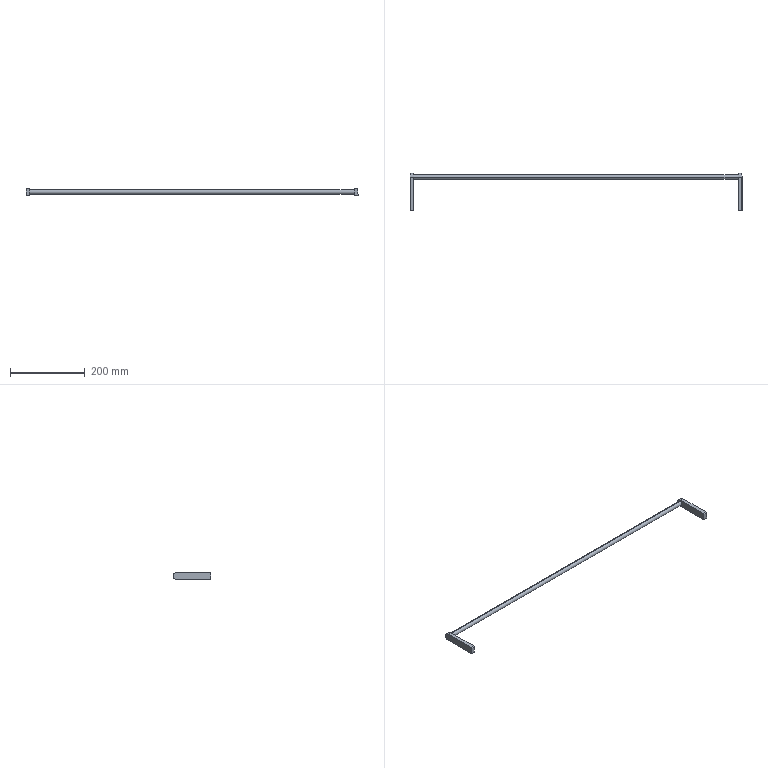Component | SolidWorks | D012-1 | 2 solids | 22 faces | box 889 x 100 x 20 mm | volume 137403 mm3 | plane 16 | cylinder 6 | commonest cylinder face diameters 12 x4 20 x2
build123d program:
from build123d import *

# Parameters (mm, degrees)
SKETCH1_W           = 100
SKETCH1_H           = 20
BOSS_EXTRUDE1_DEPTH = 10
FILLET1_RADIUS      = 10
FILLET1_LENGTH      = 10
SKETCH2_R           = 6
CUT_EXTRUDE1_DEPTH  = 2
SKETCH3_R           = 6
BOSS_EXTRUDE2_DEPTH = 871
BOSS_EXTRUDE3_START = 10
BOSS_EXTRUDE3_DEPTH = 10
CHAMFER1_SIZE       = 1
CHAMFER2_SIZE       = 1


with BuildPart() as part:
    # Sketch1 → Boss-Extrude1 (new body)
    with BuildSketch(Plane(origin=(0, 0, 0), x_dir=(1, 0, 0), z_dir=(0, 1, 0))):
        with Locations((50, 10)):
            Rectangle(SKETCH1_W, SKETCH1_H)
    extrude(amount=BOSS_EXTRUDE1_DEPTH)

    # Fillet1: full round fillet: the end face becomes a half cylinder, R = half its width
    fillet1_face = Plane((100, 5, -10), x_dir=(0, 1, 0), z_dir=(1, 0, 0))  # on the end face: x along it, z out of the body
    fillet1_slab = fillet1_face.offset(-FILLET1_RADIUS / 2) * Box(FILLET1_LENGTH, 2 * FILLET1_RADIUS, FILLET1_RADIUS, mode=Mode.PRIVATE)  # the body's end, R deep
    fillet1_round = Plane((90, 5, -10), x_dir=(1, 0, 0), z_dir=(0, 1, 0)) * Cylinder(FILLET1_RADIUS, FILLET1_LENGTH, mode=Mode.PRIVATE)  # its axis R under the face
    add(fillet1_slab - fillet1_round, mode=Mode.SUBTRACT)

    # Sketch2 → Cut-Extrude1 (cut)
    with BuildSketch(Plane(origin=(0, 10, 0), x_dir=(1, 0, 0), z_dir=(0, 1, 0))):
        with Locations(Location((90, 10, 0), (0, 0, 270))):
            Circle(SKETCH2_R)
    extrude(amount=-CUT_EXTRUDE1_DEPTH, mode=Mode.SUBTRACT)

    # Chamfer1
    chamfer1_edges = [part.edges().sort_by_distance(p)[0] for p in [
        (0, 5, -20),
        (0, 5, 0),
    ]]
    chamfer(chamfer1_edges, length=CHAMFER1_SIZE)


with BuildPart() as body_2:
    # Sketch3 → Boss-Extrude2 (new body)
    with BuildSketch(Plane(origin=(0, 8, 0), x_dir=(1, 0, 0), z_dir=(0, 1, 0))):
        with Locations(Location((90, 10, 0), (0, 0, 90))):
            Circle(SKETCH3_R)
    extrude(amount=BOSS_EXTRUDE2_DEPTH)

    # Sketch4 → Boss-Extrude3 (add)
    with BuildSketch(Plane(origin=(0, 879, 0), x_dir=(1, 0, 0), z_dir=(0, 1, 0)).offset(BOSS_EXTRUDE3_START)):
        with BuildLine():
            Line((0, 0), (90, 0))
            ThreePointArc((90, 0), (100, 10), (90, 20))
            Line((90, 20), (0, 20))
            Line((0, 20), (0, 0))
        make_face()
    extrude(amount=-BOSS_EXTRUDE3_DEPTH)

    # Chamfer2
    chamfer2_edges = [body_2.edges().sort_by_distance(p)[0] for p in [
        (0, 884, -20),
        (0, 884, 0),
    ]]
    chamfer(chamfer2_edges, length=CHAMFER2_SIZE)


solid = Compound([part.part, body_2.part])

# Placed as in the assembly
solid = solid.moved(Location((879, -35, 32.732), (0, 0, 90)))
STEP:
#1=CARTESIAN_POINT('',(-0.,2.165,1.131));
#2=VERTEX_POINT('',#1);
#3=CARTESIAN_POINT('',(-0.,2.165,0.6587));
#4=VERTEX_POINT('',#3);
#5=CARTESIAN_POINT('',(-0.,2.165,0.895));
#6=DIRECTION('',(-1.,-0.,-0.));
#7=DIRECTION('',(-0.,-0.,1.));
#8=AXIS2_PLACEMENT_3D('',#5,#6,#7);
#9=CIRCLE('',#8,0.2362);
#10=EDGE_CURVE('',#2,#4,#9,.T.);
#11=ORIENTED_EDGE('',*,*,#10,.F.);
#12=CARTESIAN_POINT('',(34.291,2.165,1.131));
#13=VERTEX_POINT('',#12);
#14=CARTESIAN_POINT('',(-0.,2.165,1.131));
#15=DIRECTION('',(1.,0.,0.));
#16=VECTOR('',#15,39.37);
#17=LINE('',#14,#16);
#18=EDGE_CURVE('',#2,#13,#17,.T.);
#19=ORIENTED_EDGE('',*,*,#18,.T.);
#20=CARTESIAN_POINT('',(34.291,2.165,0.6587));
#21=VERTEX_POINT('',#20);
#22=CARTESIAN_POINT('',(34.291,2.165,0.895));
#23=DIRECTION('',(-1.,-0.,-0.));
#24=DIRECTION('',(0.,-0.,1.));
#25=AXIS2_PLACEMENT_3D('',#22,#23,#24);
#26=CIRCLE('',#25,0.2362);
#27=EDGE_CURVE('',#13,#21,#26,.T.);
#28=ORIENTED_EDGE('',*,*,#27,.T.);
#29=CARTESIAN_POINT('',(-0.,2.165,0.6587));
#30=DIRECTION('',(1.,0.,0.));
#31=VECTOR('',#30,39.37);
#32=LINE('',#29,#31);
#33=EDGE_CURVE('',#4,#21,#32,.T.);
#34=ORIENTED_EDGE('',*,*,#33,.F.);
#35=EDGE_LOOP('',(#11,#19,#28,#34));
#36=FACE_OUTER_BOUND('',#35,.T.);
#37=CARTESIAN_POINT('',(-0.,2.165,0.895));
#38=DIRECTION('',(1.,0.,0.));
#39=DIRECTION('',(0.,0.,-1.));
#40=AXIS2_PLACEMENT_3D('',#37,#38,#39);
#41=CYLINDRICAL_SURFACE('',#40,0.2362);
#42=ADVANCED_FACE('',(#36),#41,.T.);
#43=ORIENTED_EDGE('',*,*,#18,.F.);
#44=CARTESIAN_POINT('',(-0.,2.165,0.895));
#45=DIRECTION('',(-1.,-0.,-0.));
#46=DIRECTION('',(-0.,-0.,1.));
#47=AXIS2_PLACEMENT_3D('',#44,#45,#46);
#48=CIRCLE('',#47,0.2362);
#49=EDGE_CURVE('',#4,#2,#48,.T.);
#50=ORIENTED_EDGE('',*,*,#49,.F.);
#51=ORIENTED_EDGE('',*,*,#33,.T.);
#52=CARTESIAN_POINT('',(34.291,2.165,0.895));
#53=DIRECTION('',(-1.,-0.,-0.));
#54=DIRECTION('',(0.,-0.,1.));
#55=AXIS2_PLACEMENT_3D('',#52,#53,#54);
#56=CIRCLE('',#55,0.2362);
#57=EDGE_CURVE('',#21,#13,#56,.T.);
#58=ORIENTED_EDGE('',*,*,#57,.T.);
#59=EDGE_LOOP('',(#43,#50,#51,#58));
#60=FACE_OUTER_BOUND('',#59,.T.);
#61=CARTESIAN_POINT('',(-0.,2.165,0.895));
#62=DIRECTION('',(1.,0.,0.));
#63=DIRECTION('',(0.,0.,-1.));
#64=AXIS2_PLACEMENT_3D('',#61,#62,#63);
#65=CYLINDRICAL_SURFACE('',#64,0.2362);
#66=ADVANCED_FACE('',(#60),#65,.T.);
#67=ORIENTED_EDGE('',*,*,#57,.F.);
#68=ORIENTED_EDGE('',*,*,#27,.F.);
#69=EDGE_LOOP('',(#67,#68));
#70=FACE_OUTER_BOUND('',#69,.T.);
#71=CARTESIAN_POINT('',(34.291,2.165,0.895));
#72=DIRECTION('',(-1.,-0.,-0.));
#73=DIRECTION('',(-0.,-0.,1.));
#74=AXIS2_PLACEMENT_3D('',#71,#72,#73);
#75=PLANE('',#74);
#76=ADVANCED_FACE('',(#70),#75,.F.);
#77=CARTESIAN_POINT('',(-0.,-1.378,0.5406));
#78=VERTEX_POINT('',#77);
#79=CARTESIAN_POINT('',(-0.,-1.378,1.249));
#80=VERTEX_POINT('',#79);
#81=CARTESIAN_POINT('',(-0.,-1.378,0.5013));
#82=DIRECTION('',(-0.,-0.,1.));
#83=VECTOR('',#82,39.37);
#84=LINE('',#81,#83);
#85=EDGE_CURVE('',#78,#80,#84,.T.);
#86=ORIENTED_EDGE('',*,*,#85,.T.);
#87=CARTESIAN_POINT('',(-0.3937,-1.378,1.249));
#88=VERTEX_POINT('',#87);
#89=CARTESIAN_POINT('',(-0.3937,-1.378,1.249));
#90=DIRECTION('',(-1.,-0.,-0.));
#91=VECTOR('',#90,39.37);
#92=LINE('',#89,#91);
#93=EDGE_CURVE('',#80,#88,#92,.T.);
#94=ORIENTED_EDGE('',*,*,#93,.T.);
#95=CARTESIAN_POINT('',(-0.3937,-1.378,0.5406));
#96=VERTEX_POINT('',#95);
#97=CARTESIAN_POINT('',(-0.3937,-1.378,0.5013));
#98=DIRECTION('',(-0.,-0.,1.));
#99=VECTOR('',#98,39.37);
#100=LINE('',#97,#99);
#101=EDGE_CURVE('',#96,#88,#100,.T.);
#102=ORIENTED_EDGE('',*,*,#101,.F.);
#103=CARTESIAN_POINT('',(-0.3937,-1.378,0.5406));
#104=DIRECTION('',(1.,0.,0.));
#105=VECTOR('',#104,39.37);
#106=LINE('',#103,#105);
#107=EDGE_CURVE('',#96,#78,#106,.T.);
#108=ORIENTED_EDGE('',*,*,#107,.T.);
#109=EDGE_LOOP('',(#86,#94,#102,#108));
#110=FACE_OUTER_BOUND('',#109,.T.);
#111=CARTESIAN_POINT('',(-0.3937,-1.378,0.5013));
#112=DIRECTION('',(-0.,1.,0.));
#113=DIRECTION('',(0.,0.,-1.));
#114=AXIS2_PLACEMENT_3D('',#111,#112,#113);
#115=PLANE('',#114);
#116=ADVANCED_FACE('',(#110),#115,.F.);
#117=CARTESIAN_POINT('',(-0.3937,-1.339,1.289));
#118=VERTEX_POINT('',#117);
#119=CARTESIAN_POINT('',(-0.3937,2.165,1.289));
#120=VERTEX_POINT('',#119);
#121=CARTESIAN_POINT('',(-0.3937,-1.378,1.289));
#122=DIRECTION('',(-0.,1.,0.));
#123=VECTOR('',#122,39.37);
#124=LINE('',#121,#123);
#125=EDGE_CURVE('',#118,#120,#124,.T.);
#126=ORIENTED_EDGE('',*,*,#125,.F.);
#127=CARTESIAN_POINT('',(-0.,-1.339,1.289));
#128=VERTEX_POINT('',#127);
#129=CARTESIAN_POINT('',(-0.3937,-1.339,1.289));
#130=DIRECTION('',(1.,0.,0.));
#131=VECTOR('',#130,39.37);
#132=LINE('',#129,#131);
#133=EDGE_CURVE('',#118,#128,#132,.T.);
#134=ORIENTED_EDGE('',*,*,#133,.T.);
#135=CARTESIAN_POINT('',(-0.,2.165,1.289));
#136=VERTEX_POINT('',#135);
#137=CARTESIAN_POINT('',(-0.,-1.378,1.289));
#138=DIRECTION('',(-0.,1.,0.));
#139=VECTOR('',#138,39.37);
#140=LINE('',#137,#139);
#141=EDGE_CURVE('',#128,#136,#140,.T.);
#142=ORIENTED_EDGE('',*,*,#141,.T.);
#143=CARTESIAN_POINT('',(-0.3937,2.165,1.289));
#144=DIRECTION('',(1.,0.,0.));
#145=VECTOR('',#144,39.37);
#146=LINE('',#143,#145);
#147=EDGE_CURVE('',#120,#136,#146,.T.);
#148=ORIENTED_EDGE('',*,*,#147,.F.);
#149=EDGE_LOOP('',(#126,#134,#142,#148));
#150=FACE_OUTER_BOUND('',#149,.T.);
#151=CARTESIAN_POINT('',(-0.3937,-1.378,1.289));
#152=DIRECTION('',(0.,0.,-1.));
#153=DIRECTION('',(0.,-1.,-0.));
#154=AXIS2_PLACEMENT_3D('',#151,#152,#153);
#155=PLANE('',#154);
#156=ADVANCED_FACE('',(#150),#155,.F.);
#157=CARTESIAN_POINT('',(-0.,2.165,0.5013));
#158=VERTEX_POINT('',#157);
#159=CARTESIAN_POINT('',(-0.,2.165,0.895));
#160=DIRECTION('',(-1.,-0.,-0.));
#161=DIRECTION('',(-0.,-0.,1.));
#162=AXIS2_PLACEMENT_3D('',#159,#160,#161);
#163=CIRCLE('',#162,0.3937);
#164=EDGE_CURVE('',#136,#158,#163,.T.);
#165=ORIENTED_EDGE('',*,*,#164,.T.);
#166=CARTESIAN_POINT('',(-0.3937,2.165,0.5013));
#167=VERTEX_POINT('',#166);
#168=CARTESIAN_POINT('',(-0.3937,2.165,0.5013));
#169=DIRECTION('',(1.,0.,0.));
#170=VECTOR('',#169,39.37);
#171=LINE('',#168,#170);
#172=EDGE_CURVE('',#167,#158,#171,.T.);
#173=ORIENTED_EDGE('',*,*,#172,.F.);
#174=CARTESIAN_POINT('',(-0.3937,2.165,0.895));
#175=DIRECTION('',(-1.,-0.,-0.));
#176=DIRECTION('',(-0.,-0.,1.));
#177=AXIS2_PLACEMENT_3D('',#174,#175,#176);
#178=CIRCLE('',#177,0.3937);
#179=EDGE_CURVE('',#120,#167,#178,.T.);
#180=ORIENTED_EDGE('',*,*,#179,.F.);
#181=ORIENTED_EDGE('',*,*,#147,.T.);
#182=EDGE_LOOP('',(#165,#173,#180,#181));
#183=FACE_OUTER_BOUND('',#182,.T.);
#184=CARTESIAN_POINT('',(-0.3937,2.165,0.895));
#185=DIRECTION('',(1.,0.,0.));
#186=DIRECTION('',(0.,0.,-1.));
#187=AXIS2_PLACEMENT_3D('',#184,#185,#186);
#188=CYLINDRICAL_SURFACE('',#187,0.3937);
#189=ADVANCED_FACE('',(#183),#188,.T.);
#190=CARTESIAN_POINT('',(-0.,-1.339,0.5013));
#191=VERTEX_POINT('',#190);
#192=CARTESIAN_POINT('',(-0.,2.165,0.5013));
#193=DIRECTION('',(0.,-1.,-0.));
#194=VECTOR('',#193,39.37);
#195=LINE('',#192,#194);
#196=EDGE_CURVE('',#158,#191,#195,.T.);
#197=ORIENTED_EDGE('',*,*,#196,.T.);
#198=CARTESIAN_POINT('',(-0.3937,-1.339,0.5013));
#199=VERTEX_POINT('',#198);
#200=CARTESIAN_POINT('',(-0.3937,-1.339,0.5013));
#201=DIRECTION('',(-1.,-0.,-0.));
#202=VECTOR('',#201,39.37);
#203=LINE('',#200,#202);
#204=EDGE_CURVE('',#191,#199,#203,.T.);
#205=ORIENTED_EDGE('',*,*,#204,.T.);
#206=CARTESIAN_POINT('',(-0.3937,2.165,0.5013));
#207=DIRECTION('',(0.,-1.,-0.));
#208=VECTOR('',#207,39.37);
#209=LINE('',#206,#208);
#210=EDGE_CURVE('',#167,#199,#209,.T.);
#211=ORIENTED_EDGE('',*,*,#210,.F.);
#212=ORIENTED_EDGE('',*,*,#172,.T.);
#213=EDGE_LOOP('',(#197,#205,#211,#212));
#214=FACE_OUTER_BOUND('',#213,.T.);
#215=CARTESIAN_POINT('',(-0.3937,2.165,0.5013));
#216=DIRECTION('',(-0.,-0.,1.));
#217=DIRECTION('',(-0.,1.,0.));
#218=AXIS2_PLACEMENT_3D('',#215,#216,#217);
#219=PLANE('',#218);
#220=ADVANCED_FACE('',(#214),#219,.F.);
#221=ORIENTED_EDGE('',*,*,#101,.T.);
#222=CARTESIAN_POINT('',(-0.3937,0.2165,2.844));
#223=DIRECTION('',(-0.,0.7071,0.7071));
#224=VECTOR('',#223,39.37);
#225=LINE('',#222,#224);
#226=EDGE_CURVE('',#88,#118,#225,.T.);
#227=ORIENTED_EDGE('',*,*,#226,.T.);
#228=ORIENTED_EDGE('',*,*,#125,.T.);
#229=ORIENTED_EDGE('',*,*,#179,.T.);
#230=ORIENTED_EDGE('',*,*,#210,.T.);
#231=CARTESIAN_POINT('',(-0.3937,0.2165,-1.054));
#232=DIRECTION('',(-0.,-0.7071,0.7071));
#233=VECTOR('',#232,39.37);
#234=LINE('',#231,#233);
#235=EDGE_CURVE('',#199,#96,#234,.T.);
#236=ORIENTED_EDGE('',*,*,#235,.T.);
#237=EDGE_LOOP('',(#221,#227,#228,#229,#230,#236));
#238=FACE_OUTER_BOUND('',#237,.T.);
#239=CARTESIAN_POINT('',(-0.3937,2.165,0.895));
#240=DIRECTION('',(-1.,-0.,-0.));
#241=DIRECTION('',(-0.,-0.,1.));
#242=AXIS2_PLACEMENT_3D('',#239,#240,#241);
#243=PLANE('',#242);
#244=ADVANCED_FACE('',(#238),#243,.T.);
#245=ORIENTED_EDGE('',*,*,#49,.T.);
#246=ORIENTED_EDGE('',*,*,#10,.T.);
#247=EDGE_LOOP('',(#245,#246));
#248=FACE_BOUND('',#247,.T.);
#249=ORIENTED_EDGE('',*,*,#141,.F.);
#250=CARTESIAN_POINT('',(-0.,-1.339,1.289));
#251=DIRECTION('',(0.,-0.7071,-0.7071));
#252=VECTOR('',#251,39.37);
#253=LINE('',#250,#252);
#254=EDGE_CURVE('',#128,#80,#253,.T.);
#255=ORIENTED_EDGE('',*,*,#254,.T.);
#256=ORIENTED_EDGE('',*,*,#85,.F.);
#257=CARTESIAN_POINT('',(-0.,-1.378,0.5406));
#258=DIRECTION('',(0.,0.7071,-0.7071));
#259=VECTOR('',#258,39.37);
#260=LINE('',#257,#259);
#261=EDGE_CURVE('',#78,#191,#260,.T.);
#262=ORIENTED_EDGE('',*,*,#261,.T.);
#263=ORIENTED_EDGE('',*,*,#196,.F.);
#264=ORIENTED_EDGE('',*,*,#164,.F.);
#265=EDGE_LOOP('',(#249,#255,#256,#262,#263,#264));
#266=FACE_OUTER_BOUND('',#265,.T.);
#267=CARTESIAN_POINT('',(-0.,2.165,0.895));
#268=DIRECTION('',(-1.,-0.,-0.));
#269=DIRECTION('',(-0.,-0.,1.));
#270=AXIS2_PLACEMENT_3D('',#267,#268,#269);
#271=PLANE('',#270);
#272=ADVANCED_FACE('',(#248,#266),#271,.F.);
#273=ORIENTED_EDGE('',*,*,#226,.F.);
#274=ORIENTED_EDGE('',*,*,#93,.F.);
#275=ORIENTED_EDGE('',*,*,#254,.F.);
#276=ORIENTED_EDGE('',*,*,#133,.F.);
#277=EDGE_LOOP('',(#273,#274,#275,#276));
#278=FACE_OUTER_BOUND('',#277,.T.);
#279=CARTESIAN_POINT('',(-0.3937,-1.339,1.289));
#280=DIRECTION('',(0.,0.7071,-0.7071));
#281=DIRECTION('',(1.,0.,0.));
#282=AXIS2_PLACEMENT_3D('',#279,#280,#281);
#283=PLANE('',#282);
#284=ADVANCED_FACE('',(#278),#283,.F.);
#285=ORIENTED_EDGE('',*,*,#235,.F.);
#286=ORIENTED_EDGE('',*,*,#204,.F.);
#287=ORIENTED_EDGE('',*,*,#261,.F.);
#288=ORIENTED_EDGE('',*,*,#107,.F.);
#289=EDGE_LOOP('',(#285,#286,#287,#288));
#290=FACE_OUTER_BOUND('',#289,.T.);
#291=CARTESIAN_POINT('',(-0.3937,-1.378,0.5406));
#292=DIRECTION('',(-0.,0.7071,0.7071));
#293=DIRECTION('',(1.,0.,0.));
#294=AXIS2_PLACEMENT_3D('',#291,#292,#293);
#295=PLANE('',#294);
#296=ADVANCED_FACE('',(#290),#295,.F.);
#297=CLOSED_SHELL('',(#42,#66,#76,#116,#156,#189,#220,#244,#272,#284,#296));
#298=MANIFOLD_SOLID_BREP('',#297);
#299=CARTESIAN_POINT('',(34.291,2.165,0.6587));
#300=VERTEX_POINT('',#299);
#301=CARTESIAN_POINT('',(34.291,2.165,1.131));
#302=VERTEX_POINT('',#301);
#303=CARTESIAN_POINT('',(34.291,2.165,0.895));
#304=DIRECTION('',(-1.,-0.,-0.));
#305=DIRECTION('',(0.,-0.,1.));
#306=AXIS2_PLACEMENT_3D('',#303,#304,#305);
#307=CIRCLE('',#306,0.2362);
#308=EDGE_CURVE('',#300,#302,#307,.T.);
#309=ORIENTED_EDGE('',*,*,#308,.F.);
#310=CARTESIAN_POINT('',(34.213,2.165,0.6587));
#311=VERTEX_POINT('',#310);
#312=CARTESIAN_POINT('',(34.291,2.165,0.6587));
#313=DIRECTION('',(-1.,-0.,-0.));
#314=VECTOR('',#313,39.37);
#315=LINE('',#312,#314);
#316=EDGE_CURVE('',#300,#311,#315,.T.);
#317=ORIENTED_EDGE('',*,*,#316,.T.);
#318=CARTESIAN_POINT('',(34.213,2.165,1.131));
#319=VERTEX_POINT('',#318);
#320=CARTESIAN_POINT('',(34.213,2.165,0.895));
#321=DIRECTION('',(-1.,-0.,-0.));
#322=DIRECTION('',(0.,-0.,1.));
#323=AXIS2_PLACEMENT_3D('',#320,#321,#322);
#324=CIRCLE('',#323,0.2362);
#325=EDGE_CURVE('',#311,#319,#324,.T.);
#326=ORIENTED_EDGE('',*,*,#325,.T.);
#327=CARTESIAN_POINT('',(34.291,2.165,1.131));
#328=DIRECTION('',(-1.,-0.,-0.));
#329=VECTOR('',#328,39.37);
#330=LINE('',#327,#329);
#331=EDGE_CURVE('',#302,#319,#330,.T.);
#332=ORIENTED_EDGE('',*,*,#331,.F.);
#333=EDGE_LOOP('',(#309,#317,#326,#332));
#334=FACE_OUTER_BOUND('',#333,.T.);
#335=CARTESIAN_POINT('',(34.291,2.165,0.895));
#336=DIRECTION('',(-1.,-0.,-0.));
#337=DIRECTION('',(0.,-0.,1.));
#338=AXIS2_PLACEMENT_3D('',#335,#336,#337);
#339=CYLINDRICAL_SURFACE('',#338,0.2362);
#340=ADVANCED_FACE('',(#334),#339,.F.);
#341=CARTESIAN_POINT('',(34.606,2.165,1.289));
#342=VERTEX_POINT('',#341);
#343=CARTESIAN_POINT('',(34.213,2.165,1.289));
#344=VERTEX_POINT('',#343);
#345=CARTESIAN_POINT('',(34.213,2.165,1.289));
#346=DIRECTION('',(-1.,-0.,-0.));
#347=VECTOR('',#346,39.37);
#348=LINE('',#345,#347);
#349=EDGE_CURVE('',#342,#344,#348,.T.);
#350=ORIENTED_EDGE('',*,*,#349,.F.);
#351=CARTESIAN_POINT('',(34.606,2.165,0.5013));
#352=VERTEX_POINT('',#351);
#353=CARTESIAN_POINT('',(34.606,2.165,0.895));
#354=DIRECTION('',(1.,0.,0.));
#355=DIRECTION('',(0.,0.,-1.));
#356=AXIS2_PLACEMENT_3D('',#353,#354,#355);
#357=CIRCLE('',#356,0.3937);
#358=EDGE_CURVE('',#352,#342,#357,.T.);
#359=ORIENTED_EDGE('',*,*,#358,.F.);
#360=CARTESIAN_POINT('',(34.213,2.165,0.5013));
#361=VERTEX_POINT('',#360);
#362=CARTESIAN_POINT('',(34.213,2.165,0.5013));
#363=DIRECTION('',(1.,0.,0.));
#364=VECTOR('',#363,39.37);
#365=LINE('',#362,#364);
#366=EDGE_CURVE('',#361,#352,#365,.T.);
#367=ORIENTED_EDGE('',*,*,#366,.F.);
#368=CARTESIAN_POINT('',(34.213,2.165,0.895));
#369=DIRECTION('',(-1.,-0.,-0.));
#370=DIRECTION('',(0.,0.,-1.));
#371=AXIS2_PLACEMENT_3D('',#368,#369,#370);
#372=CIRCLE('',#371,0.3937);
#373=EDGE_CURVE('',#344,#361,#372,.T.);
#374=ORIENTED_EDGE('',*,*,#373,.F.);
#375=EDGE_LOOP('',(#350,#359,#367,#374));
#376=FACE_OUTER_BOUND('',#375,.T.);
#377=CARTESIAN_POINT('',(34.606,2.165,0.895));
#378=DIRECTION('',(1.,0.,0.));
#379=DIRECTION('',(0.,0.,-1.));
#380=AXIS2_PLACEMENT_3D('',#377,#378,#379);
#381=CYLINDRICAL_SURFACE('',#380,0.3937);
#382=ADVANCED_FACE('',(#376),#381,.T.);
#383=CARTESIAN_POINT('',(34.606,-1.378,0.5406));
#384=VERTEX_POINT('',#383);
#385=CARTESIAN_POINT('',(34.606,-1.378,1.249));
#386=VERTEX_POINT('',#385);
#387=CARTESIAN_POINT('',(34.606,-1.378,1.289));
#388=DIRECTION('',(-0.,-0.,1.));
#389=VECTOR('',#388,39.37);
#390=LINE('',#387,#389);
#391=EDGE_CURVE('',#384,#386,#390,.T.);
#392=ORIENTED_EDGE('',*,*,#391,.T.);
#393=CARTESIAN_POINT('',(34.213,-1.378,1.249));
#394=VERTEX_POINT('',#393);
#395=CARTESIAN_POINT('',(34.213,-1.378,1.249));
#396=DIRECTION('',(-1.,-0.,-0.));
#397=VECTOR('',#396,39.37);
#398=LINE('',#395,#397);
#399=EDGE_CURVE('',#386,#394,#398,.T.);
#400=ORIENTED_EDGE('',*,*,#399,.T.);
#401=CARTESIAN_POINT('',(34.213,-1.378,0.5406));
#402=VERTEX_POINT('',#401);
#403=CARTESIAN_POINT('',(34.213,-1.378,1.289));
#404=DIRECTION('',(-0.,-0.,1.));
#405=VECTOR('',#404,39.37);
#406=LINE('',#403,#405);
#407=EDGE_CURVE('',#402,#394,#406,.T.);
#408=ORIENTED_EDGE('',*,*,#407,.F.);
#409=CARTESIAN_POINT('',(34.213,-1.378,0.5406));
#410=DIRECTION('',(1.,0.,0.));
#411=VECTOR('',#410,39.37);
#412=LINE('',#409,#411);
#413=EDGE_CURVE('',#402,#384,#412,.T.);
#414=ORIENTED_EDGE('',*,*,#413,.T.);
#415=EDGE_LOOP('',(#392,#400,#408,#414));
#416=FACE_OUTER_BOUND('',#415,.T.);
#417=CARTESIAN_POINT('',(34.213,-1.378,1.289));
#418=DIRECTION('',(-0.,1.,0.));
#419=DIRECTION('',(0.,0.,-1.));
#420=AXIS2_PLACEMENT_3D('',#417,#418,#419);
#421=PLANE('',#420);
#422=ADVANCED_FACE('',(#416),#421,.F.);
#423=CARTESIAN_POINT('',(34.213,-1.339,1.289));
#424=VERTEX_POINT('',#423);
#425=CARTESIAN_POINT('',(34.213,-1.378,1.289));
#426=DIRECTION('',(-0.,1.,0.));
#427=VECTOR('',#426,39.37);
#428=LINE('',#425,#427);
#429=EDGE_CURVE('',#424,#344,#428,.T.);
#430=ORIENTED_EDGE('',*,*,#429,.F.);
#431=CARTESIAN_POINT('',(34.606,-1.339,1.289));
#432=VERTEX_POINT('',#431);
#433=CARTESIAN_POINT('',(34.213,-1.339,1.289));
#434=DIRECTION('',(1.,0.,0.));
#435=VECTOR('',#434,39.37);
#436=LINE('',#433,#435);
#437=EDGE_CURVE('',#424,#432,#436,.T.);
#438=ORIENTED_EDGE('',*,*,#437,.T.);
#439=CARTESIAN_POINT('',(34.606,-1.378,1.289));
#440=DIRECTION('',(-0.,1.,0.));
#441=VECTOR('',#440,39.37);
#442=LINE('',#439,#441);
#443=EDGE_CURVE('',#432,#342,#442,.T.);
#444=ORIENTED_EDGE('',*,*,#443,.T.);
#445=ORIENTED_EDGE('',*,*,#349,.T.);
#446=EDGE_LOOP('',(#430,#438,#444,#445));
#447=FACE_OUTER_BOUND('',#446,.T.);
#448=CARTESIAN_POINT('',(34.213,-1.378,1.289));
#449=DIRECTION('',(0.,0.,-1.));
#450=DIRECTION('',(0.,-1.,-0.));
#451=AXIS2_PLACEMENT_3D('',#448,#449,#450);
#452=PLANE('',#451);
#453=ADVANCED_FACE('',(#447),#452,.F.);
#454=CARTESIAN_POINT('',(34.606,-1.339,0.5013));
#455=VERTEX_POINT('',#454);
#456=CARTESIAN_POINT('',(34.606,-1.378,0.5013));
#457=DIRECTION('',(0.,-1.,-0.));
#458=VECTOR('',#457,39.37);
#459=LINE('',#456,#458);
#460=EDGE_CURVE('',#352,#455,#459,.T.);
#461=ORIENTED_EDGE('',*,*,#460,.T.);
#462=CARTESIAN_POINT('',(34.213,-1.339,0.5013));
#463=VERTEX_POINT('',#462);
#464=CARTESIAN_POINT('',(34.213,-1.339,0.5013));
#465=DIRECTION('',(-1.,-0.,-0.));
#466=VECTOR('',#465,39.37);
#467=LINE('',#464,#466);
#468=EDGE_CURVE('',#455,#463,#467,.T.);
#469=ORIENTED_EDGE('',*,*,#468,.T.);
#470=CARTESIAN_POINT('',(34.213,-1.378,0.5013));
#471=DIRECTION('',(0.,-1.,-0.));
#472=VECTOR('',#471,39.37);
#473=LINE('',#470,#472);
#474=EDGE_CURVE('',#361,#463,#473,.T.);
#475=ORIENTED_EDGE('',*,*,#474,.F.);
#476=ORIENTED_EDGE('',*,*,#366,.T.);
#477=EDGE_LOOP('',(#461,#469,#475,#476));
#478=FACE_OUTER_BOUND('',#477,.T.);
#479=CARTESIAN_POINT('',(34.213,-1.378,0.5013));
#480=DIRECTION('',(-0.,-0.,1.));
#481=DIRECTION('',(-0.,1.,0.));
#482=AXIS2_PLACEMENT_3D('',#479,#480,#481);
#483=PLANE('',#482);
#484=ADVANCED_FACE('',(#478),#483,.F.);
#485=CARTESIAN_POINT('',(34.213,2.165,0.895));
#486=DIRECTION('',(-1.,-0.,-0.));
#487=DIRECTION('',(0.,-0.,1.));
#488=AXIS2_PLACEMENT_3D('',#485,#486,#487);
#489=CIRCLE('',#488,0.2362);
#490=EDGE_CURVE('',#319,#311,#489,.T.);
#491=ORIENTED_EDGE('',*,*,#490,.F.);
#492=ORIENTED_EDGE('',*,*,#325,.F.);
#493=EDGE_LOOP('',(#491,#492));
#494=FACE_BOUND('',#493,.T.);
#495=ORIENTED_EDGE('',*,*,#407,.T.);
#496=CARTESIAN_POINT('',(34.213,-1.339,1.289));
#497=DIRECTION('',(-0.,0.7071,0.7071));
#498=VECTOR('',#497,39.37);
#499=LINE('',#496,#498);
#500=EDGE_CURVE('',#394,#424,#499,.T.);
#501=ORIENTED_EDGE('',*,*,#500,.T.);
#502=ORIENTED_EDGE('',*,*,#429,.T.);
#503=ORIENTED_EDGE('',*,*,#373,.T.);
#504=ORIENTED_EDGE('',*,*,#474,.T.);
#505=CARTESIAN_POINT('',(34.213,-1.378,0.5406));
#506=DIRECTION('',(-0.,-0.7071,0.7071));
#507=VECTOR('',#506,39.37);
#508=LINE('',#505,#507);
#509=EDGE_CURVE('',#463,#402,#508,.T.);
#510=ORIENTED_EDGE('',*,*,#509,.T.);
#511=EDGE_LOOP('',(#495,#501,#502,#503,#504,#510));
#512=FACE_OUTER_BOUND('',#511,.T.);
#513=CARTESIAN_POINT('',(34.213,-1.378,1.289));
#514=DIRECTION('',(1.,0.,0.));
#515=DIRECTION('',(0.,0.,-1.));
#516=AXIS2_PLACEMENT_3D('',#513,#514,#515);
#517=PLANE('',#516);
#518=ADVANCED_FACE('',(#494,#512),#517,.F.);
#519=ORIENTED_EDGE('',*,*,#443,.F.);
#520=CARTESIAN_POINT('',(34.606,-1.358,1.269));
#521=DIRECTION('',(0.,-0.7071,-0.7071));
#522=VECTOR('',#521,39.37);
#523=LINE('',#520,#522);
#524=EDGE_CURVE('',#432,#386,#523,.T.);
#525=ORIENTED_EDGE('',*,*,#524,.T.);
#526=ORIENTED_EDGE('',*,*,#391,.F.);
#527=CARTESIAN_POINT('',(34.606,-1.752,0.9146));
#528=DIRECTION('',(0.,0.7071,-0.7071));
#529=VECTOR('',#528,39.37);
#530=LINE('',#527,#529);
#531=EDGE_CURVE('',#384,#455,#530,.T.);
#532=ORIENTED_EDGE('',*,*,#531,.T.);
#533=ORIENTED_EDGE('',*,*,#460,.F.);
#534=ORIENTED_EDGE('',*,*,#358,.T.);
#535=EDGE_LOOP('',(#519,#525,#526,#532,#533,#534));
#536=FACE_OUTER_BOUND('',#535,.T.);
#537=CARTESIAN_POINT('',(34.606,-1.378,1.289));
#538=DIRECTION('',(1.,0.,0.));
#539=DIRECTION('',(0.,0.,-1.));
#540=AXIS2_PLACEMENT_3D('',#537,#538,#539);
#541=PLANE('',#540);
#542=ADVANCED_FACE('',(#536),#541,.T.);
#543=ORIENTED_EDGE('',*,*,#316,.F.);
#544=CARTESIAN_POINT('',(34.291,2.165,0.895));
#545=DIRECTION('',(-1.,-0.,-0.));
#546=DIRECTION('',(0.,-0.,1.));
#547=AXIS2_PLACEMENT_3D('',#544,#545,#546);
#548=CIRCLE('',#547,0.2362);
#549=EDGE_CURVE('',#302,#300,#548,.T.);
#550=ORIENTED_EDGE('',*,*,#549,.F.);
#551=ORIENTED_EDGE('',*,*,#331,.T.);
#552=ORIENTED_EDGE('',*,*,#490,.T.);
#553=EDGE_LOOP('',(#543,#550,#551,#552));
#554=FACE_OUTER_BOUND('',#553,.T.);
#555=CARTESIAN_POINT('',(34.291,2.165,0.895));
#556=DIRECTION('',(-1.,-0.,-0.));
#557=DIRECTION('',(0.,-0.,1.));
#558=AXIS2_PLACEMENT_3D('',#555,#556,#557);
#559=CYLINDRICAL_SURFACE('',#558,0.2362);
#560=ADVANCED_FACE('',(#554),#559,.F.);
#561=ORIENTED_EDGE('',*,*,#549,.T.);
#562=ORIENTED_EDGE('',*,*,#308,.T.);
#563=EDGE_LOOP('',(#561,#562));
#564=FACE_OUTER_BOUND('',#563,.T.);
#565=CARTESIAN_POINT('',(34.291,2.165,0.895));
#566=DIRECTION('',(-1.,-0.,-0.));
#567=DIRECTION('',(-0.,-0.,1.));
#568=AXIS2_PLACEMENT_3D('',#565,#566,#567);
#569=PLANE('',#568);
#570=ADVANCED_FACE('',(#564),#569,.T.);
#571=ORIENTED_EDGE('',*,*,#500,.F.);
#572=ORIENTED_EDGE('',*,*,#399,.F.);
#573=ORIENTED_EDGE('',*,*,#524,.F.);
#574=ORIENTED_EDGE('',*,*,#437,.F.);
#575=EDGE_LOOP('',(#571,#572,#573,#574));
#576=FACE_OUTER_BOUND('',#575,.T.);
#577=CARTESIAN_POINT('',(34.213,-1.339,1.289));
#578=DIRECTION('',(0.,0.7071,-0.7071));
#579=DIRECTION('',(1.,0.,0.));
#580=AXIS2_PLACEMENT_3D('',#577,#578,#579);
#581=PLANE('',#580);
#582=ADVANCED_FACE('',(#576),#581,.F.);
#583=ORIENTED_EDGE('',*,*,#509,.F.);
#584=ORIENTED_EDGE('',*,*,#468,.F.);
#585=ORIENTED_EDGE('',*,*,#531,.F.);
#586=ORIENTED_EDGE('',*,*,#413,.F.);
#587=EDGE_LOOP('',(#583,#584,#585,#586));
#588=FACE_OUTER_BOUND('',#587,.T.);
#589=CARTESIAN_POINT('',(34.213,-1.378,0.5406));
#590=DIRECTION('',(-0.,0.7071,0.7071));
#591=DIRECTION('',(1.,0.,0.));
#592=AXIS2_PLACEMENT_3D('',#589,#590,#591);
#593=PLANE('',#592);
#594=ADVANCED_FACE('',(#588),#593,.F.);
#595=CLOSED_SHELL('',(#340,#382,#422,#453,#484,#518,#542,#560,#570,#582,#594));
#596=MANIFOLD_SOLID_BREP('',#595);
#597=CARTESIAN_POINT('',(0.,0.,0.));
#598=DIRECTION('',(0.,0.,1.));
#599=DIRECTION('',(1.,0.,0.));
#600=AXIS2_PLACEMENT_3D('',#597,#598,#599);
#601=(LENGTH_UNIT()NAMED_UNIT(*)SI_UNIT($,.METRE.));
#602=LENGTH_MEASURE_WITH_UNIT(LENGTH_MEASURE(0.0254),#601);
#603=DIMENSIONAL_EXPONENTS(1.,0.,0.,0.,0.,0.,0.);
#604=(CONVERSION_BASED_UNIT('',#602)LENGTH_UNIT()NAMED_UNIT(#603));
#605=UNCERTAINTY_MEASURE_WITH_UNIT(LENGTH_MEASURE(0.00001),#604,'','');
#606=(NAMED_UNIT(*)PLANE_ANGLE_UNIT()SI_UNIT($,.RADIAN.));
#607=(NAMED_UNIT(*)SI_UNIT($,.STERADIAN.)SOLID_ANGLE_UNIT());
#608=(GEOMETRIC_REPRESENTATION_CONTEXT(3)GLOBAL_UNCERTAINTY_ASSIGNED_CONTEXT((#605))GLOBAL_UNIT_ASSIGNED_CONTEXT((#604,#606,#607))REPRESENTATION_CONTEXT('',''));
#609=ADVANCED_BREP_SHAPE_REPRESENTATION('',(#298,#596,#600),#608);
#610=COLOUR_RGB('',0.7922,0.8196,0.9333);
#611=FILL_AREA_STYLE_COLOUR('',#610);
#612=FILL_AREA_STYLE('',(#611));
#613=SURFACE_STYLE_FILL_AREA(#612);
#614=SURFACE_SIDE_STYLE('',(#613));
#615=SURFACE_STYLE_USAGE(.BOTH.,#614);
#616=PRESENTATION_STYLE_ASSIGNMENT((#615));
#617=STYLED_ITEM('',(#616),#298);
#618=(LENGTH_UNIT()NAMED_UNIT(*)SI_UNIT($,.METRE.));
#619=LENGTH_MEASURE_WITH_UNIT(LENGTH_MEASURE(0.0254),#618);
#620=DIMENSIONAL_EXPONENTS(1.,0.,0.,0.,0.,0.,0.);
#621=(CONVERSION_BASED_UNIT('',#619)LENGTH_UNIT()NAMED_UNIT(#620));
#622=UNCERTAINTY_MEASURE_WITH_UNIT(LENGTH_MEASURE(0.00001),#621,'','');
#623=(NAMED_UNIT(*)PLANE_ANGLE_UNIT()SI_UNIT($,.RADIAN.));
#624=(NAMED_UNIT(*)SI_UNIT($,.STERADIAN.)SOLID_ANGLE_UNIT());
#625=(GEOMETRIC_REPRESENTATION_CONTEXT(3)GLOBAL_UNCERTAINTY_ASSIGNED_CONTEXT((#622))GLOBAL_UNIT_ASSIGNED_CONTEXT((#621,#623,#624))REPRESENTATION_CONTEXT('',''));
#626=MECHANICAL_DESIGN_GEOMETRIC_PRESENTATION_REPRESENTATION('',(#617),#625);
#627=COLOUR_RGB('',0.7922,0.8196,0.9333);
#628=FILL_AREA_STYLE_COLOUR('',#627);
#629=FILL_AREA_STYLE('',(#628));
#630=SURFACE_STYLE_FILL_AREA(#629);
#631=SURFACE_SIDE_STYLE('',(#630));
#632=SURFACE_STYLE_USAGE(.BOTH.,#631);
#633=PRESENTATION_STYLE_ASSIGNMENT((#632));
#634=STYLED_ITEM('',(#633),#596);
#635=PRESENTATION_LAYER_ASSIGNMENT('','',(#634));
#636=PRESENTATION_LAYER_ASSIGNMENT('','',(#617));
#637=(LENGTH_UNIT()NAMED_UNIT(*)SI_UNIT($,.METRE.));
#638=LENGTH_MEASURE_WITH_UNIT(LENGTH_MEASURE(0.0254),#637);
#639=DIMENSIONAL_EXPONENTS(1.,0.,0.,0.,0.,0.,0.);
#640=(CONVERSION_BASED_UNIT('',#638)LENGTH_UNIT()NAMED_UNIT(#639));
#641=UNCERTAINTY_MEASURE_WITH_UNIT(LENGTH_MEASURE(0.00001),#640,'','');
#642=(NAMED_UNIT(*)PLANE_ANGLE_UNIT()SI_UNIT($,.RADIAN.));
#643=(NAMED_UNIT(*)SI_UNIT($,.STERADIAN.)SOLID_ANGLE_UNIT());
#644=(GEOMETRIC_REPRESENTATION_CONTEXT(3)GLOBAL_UNCERTAINTY_ASSIGNED_CONTEXT((#641))GLOBAL_UNIT_ASSIGNED_CONTEXT((#640,#642,#643))REPRESENTATION_CONTEXT('',''));
#645=MECHANICAL_DESIGN_GEOMETRIC_PRESENTATION_REPRESENTATION('',(#634),#644);